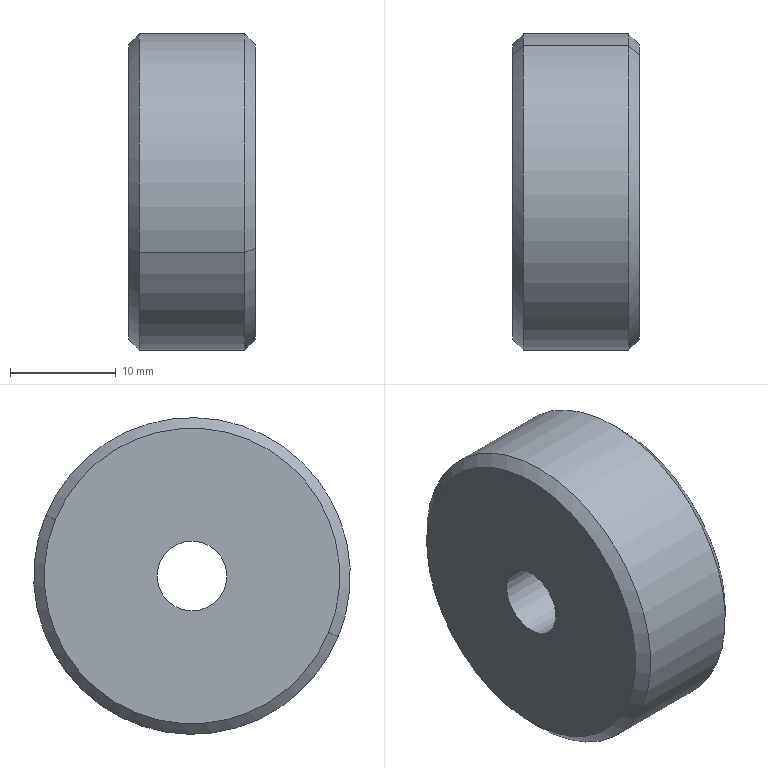Component | SolidWorks | JJDJR-3060-E-005-1 | 1 solid | 13 faces | box 12 x 30 x 30 mm | volume 7427 mm3 | cylinder 6 | cone 4 | plane 3 | commonest cylinder face diameters 12 x2 6.6 x2 30 x2 | material Tungsten Alloy
build123d program:
from build123d import *

# Parameters (mm, degrees)
SKETCH1_W                                           = 12
SKETCH1_H                                           = 15
CHAMFER1_SIZE                                       = 1
CYLINDRICAL_COUNTERSUNK_HOLE_FOR_M6_HEX_D           = 6.6
CYLINDRICAL_COUNTERSUNK_HOLE_FOR_M6_HEX_CBORE_D     = 12
CYLINDRICAL_COUNTERSUNK_HOLE_FOR_M6_HEX_CBORE_DEPTH = 7


with BuildPart() as part:
    # Sketch1 → Revolve1 (revolve)
    with BuildSketch(Plane.XY, mode=Mode.PRIVATE) as revolve1_sk:
        with Locations((6, 7.5)):
            Rectangle(SKETCH1_W, SKETCH1_H)
    revolve(revolve1_sk.sketch.rotate(Axis((-79.76, 0, 0), (1, 0, 0)), 90), axis=Axis((-79.76, 0, 0), (1, 0, 0)))

    # Chamfer1
    chamfer1_edges = [part.edges().sort_by_distance(p)[0] for p in [
        (0, 0, -15),
        (12, 0, -15),
    ]]
    chamfer(chamfer1_edges, length=CHAMFER1_SIZE)

    # Cylindrical Countersunk Hole for M6 Hex (through all)
    with Locations(Plane.ZY):
        with Locations((0, 0)):
            CounterBoreHole(CYLINDRICAL_COUNTERSUNK_HOLE_FOR_M6_HEX_D / 2, CYLINDRICAL_COUNTERSUNK_HOLE_FOR_M6_HEX_CBORE_D / 2, CYLINDRICAL_COUNTERSUNK_HOLE_FOR_M6_HEX_CBORE_DEPTH)


solid = part.part

# Placed as in the assembly
solid = solid.moved(Location((113.41, -29.263, -16.52), (-180, 0, 180)))
STEP:
#1=COLOUR_RGB('',0.7922,0.8196,0.9333);
#2=FILL_AREA_STYLE_COLOUR('',#1);
#3=FILL_AREA_STYLE('',(#2));
#4=SURFACE_STYLE_FILL_AREA(#3);
#5=SURFACE_SIDE_STYLE('',(#4));
#6=SURFACE_STYLE_USAGE(.BOTH.,#5);
#7=PRESENTATION_STYLE_ASSIGNMENT((#6));
#8=CARTESIAN_POINT('',(4.189,-1.37,-0.7406));
#9=VERTEX_POINT('',#8);
#10=CARTESIAN_POINT('',(4.189,-0.9338,-0.5602));
#11=VERTEX_POINT('',#10);
#12=CARTESIAN_POINT('',(4.189,-1.152,-0.6504));
#13=DIRECTION('',(1.,0.,0.));
#14=DIRECTION('',(0.,0.9242,0.3818));
#15=AXIS2_PLACEMENT_3D('',#12,#13,#14);
#16=CIRCLE('',#15,0.2362);
#17=EDGE_CURVE('',#9,#11,#16,.T.);
#18=ORIENTED_EDGE('',*,*,#17,.F.);
#19=CARTESIAN_POINT('',(4.465,-1.37,-0.7406));
#20=VERTEX_POINT('',#19);
#21=CARTESIAN_POINT('',(4.465,-1.37,-0.7406));
#22=DIRECTION('',(1.,0.,0.));
#23=VECTOR('',#22,39.37);
#24=LINE('',#21,#23);
#25=EDGE_CURVE('',#9,#20,#24,.T.);
#26=ORIENTED_EDGE('',*,*,#25,.T.);
#27=CARTESIAN_POINT('',(4.465,-0.9338,-0.5602));
#28=VERTEX_POINT('',#27);
#29=CARTESIAN_POINT('',(4.465,-1.152,-0.6504));
#30=DIRECTION('',(1.,0.,0.));
#31=DIRECTION('',(0.,0.9242,0.3818));
#32=AXIS2_PLACEMENT_3D('',#29,#30,#31);
#33=CIRCLE('',#32,0.2362);
#34=EDGE_CURVE('',#20,#28,#33,.T.);
#35=ORIENTED_EDGE('',*,*,#34,.T.);
#36=CARTESIAN_POINT('',(4.465,-0.9338,-0.5602));
#37=DIRECTION('',(1.,0.,0.));
#38=VECTOR('',#37,39.37);
#39=LINE('',#36,#38);
#40=EDGE_CURVE('',#11,#28,#39,.T.);
#41=ORIENTED_EDGE('',*,*,#40,.F.);
#42=EDGE_LOOP('',(#18,#26,#35,#41));
#43=FACE_OUTER_BOUND('',#42,.T.);
#44=CARTESIAN_POINT('',(4.465,-1.152,-0.6504));
#45=DIRECTION('',(1.,0.,0.));
#46=DIRECTION('',(0.,0.9242,0.3818));
#47=AXIS2_PLACEMENT_3D('',#44,#45,#46);
#48=CYLINDRICAL_SURFACE('',#47,0.2362);
#49=ADVANCED_FACE('',(#43),#48,.F.);
#50=CARTESIAN_POINT('',(3.993,-1.272,-0.7));
#51=VERTEX_POINT('',#50);
#52=CARTESIAN_POINT('',(3.993,-1.032,-0.6008));
#53=VERTEX_POINT('',#52);
#54=CARTESIAN_POINT('',(3.993,-1.152,-0.6504));
#55=DIRECTION('',(1.,0.,0.));
#56=DIRECTION('',(0.,0.9242,0.3818));
#57=AXIS2_PLACEMENT_3D('',#54,#55,#56);
#58=CIRCLE('',#57,0.1299);
#59=EDGE_CURVE('',#51,#53,#58,.T.);
#60=ORIENTED_EDGE('',*,*,#59,.F.);
#61=CARTESIAN_POINT('',(4.189,-1.272,-0.7));
#62=VERTEX_POINT('',#61);
#63=CARTESIAN_POINT('',(4.465,-1.272,-0.7));
#64=DIRECTION('',(1.,0.,0.));
#65=VECTOR('',#64,39.37);
#66=LINE('',#63,#65);
#67=EDGE_CURVE('',#51,#62,#66,.T.);
#68=ORIENTED_EDGE('',*,*,#67,.T.);
#69=CARTESIAN_POINT('',(4.189,-1.032,-0.6008));
#70=VERTEX_POINT('',#69);
#71=CARTESIAN_POINT('',(4.189,-1.152,-0.6504));
#72=DIRECTION('',(1.,0.,0.));
#73=DIRECTION('',(0.,0.9242,0.3818));
#74=AXIS2_PLACEMENT_3D('',#71,#72,#73);
#75=CIRCLE('',#74,0.1299);
#76=EDGE_CURVE('',#62,#70,#75,.T.);
#77=ORIENTED_EDGE('',*,*,#76,.T.);
#78=CARTESIAN_POINT('',(4.465,-1.032,-0.6008));
#79=DIRECTION('',(1.,0.,0.));
#80=VECTOR('',#79,39.37);
#81=LINE('',#78,#80);
#82=EDGE_CURVE('',#53,#70,#81,.T.);
#83=ORIENTED_EDGE('',*,*,#82,.F.);
#84=EDGE_LOOP('',(#60,#68,#77,#83));
#85=FACE_OUTER_BOUND('',#84,.T.);
#86=CARTESIAN_POINT('',(4.465,-1.152,-0.6504));
#87=DIRECTION('',(1.,0.,0.));
#88=DIRECTION('',(0.,0.9242,0.3818));
#89=AXIS2_PLACEMENT_3D('',#86,#87,#88);
#90=CYLINDRICAL_SURFACE('',#89,0.1299);
#91=ADVANCED_FACE('',(#85),#90,.F.);
#92=CARTESIAN_POINT('',(4.465,-0.6427,-0.4399));
#93=VERTEX_POINT('',#92);
#94=CARTESIAN_POINT('',(4.465,-1.661,-0.8609));
#95=VERTEX_POINT('',#94);
#96=CARTESIAN_POINT('',(4.465,-1.152,-0.6504));
#97=DIRECTION('',(1.,0.,0.));
#98=DIRECTION('',(0.,-0.9242,-0.3818));
#99=AXIS2_PLACEMENT_3D('',#96,#97,#98);
#100=CIRCLE('',#99,0.5512);
#101=EDGE_CURVE('',#93,#95,#100,.T.);
#102=ORIENTED_EDGE('',*,*,#101,.F.);
#103=CARTESIAN_POINT('',(4.426,-0.6063,-0.4249));
#104=VERTEX_POINT('',#103);
#105=CARTESIAN_POINT('',(4.465,-0.6427,-0.4399));
#106=DIRECTION('',(-0.7071,0.6535,0.27));
#107=VECTOR('',#106,39.37);
#108=LINE('',#105,#107);
#109=EDGE_CURVE('',#93,#104,#108,.T.);
#110=ORIENTED_EDGE('',*,*,#109,.T.);
#111=CARTESIAN_POINT('',(4.426,-1.698,-0.8759));
#112=VERTEX_POINT('',#111);
#113=CARTESIAN_POINT('',(4.426,-1.152,-0.6504));
#114=DIRECTION('',(-1.,0.,0.));
#115=DIRECTION('',(0.,-0.9242,-0.3818));
#116=AXIS2_PLACEMENT_3D('',#113,#114,#115);
#117=CIRCLE('',#116,0.5906);
#118=EDGE_CURVE('',#112,#104,#117,.T.);
#119=ORIENTED_EDGE('',*,*,#118,.F.);
#120=CARTESIAN_POINT('',(4.465,-1.661,-0.8609));
#121=DIRECTION('',(-0.7071,-0.6535,-0.27));
#122=VECTOR('',#121,39.37);
#123=LINE('',#120,#122);
#124=EDGE_CURVE('',#95,#112,#123,.T.);
#125=ORIENTED_EDGE('',*,*,#124,.F.);
#126=EDGE_LOOP('',(#102,#110,#119,#125));
#127=FACE_OUTER_BOUND('',#126,.T.);
#128=CARTESIAN_POINT('',(4.465,-1.152,-0.6504));
#129=DIRECTION('',(-1.,0.,0.));
#130=DIRECTION('',(0.,-0.9242,-0.3818));
#131=AXIS2_PLACEMENT_3D('',#128,#129,#130);
#132=CONICAL_SURFACE('',#131,0.5512,0.7854);
#133=ADVANCED_FACE('',(#127),#132,.T.);
#134=CARTESIAN_POINT('',(3.993,-1.661,-0.8609));
#135=VERTEX_POINT('',#134);
#136=CARTESIAN_POINT('',(3.993,-0.6427,-0.4399));
#137=VERTEX_POINT('',#136);
#138=CARTESIAN_POINT('',(3.993,-1.152,-0.6504));
#139=DIRECTION('',(-1.,0.,0.));
#140=DIRECTION('',(0.,0.9242,0.3818));
#141=AXIS2_PLACEMENT_3D('',#138,#139,#140);
#142=CIRCLE('',#141,0.5512);
#143=EDGE_CURVE('',#135,#137,#142,.T.);
#144=ORIENTED_EDGE('',*,*,#143,.F.);
#145=CARTESIAN_POINT('',(4.032,-1.698,-0.8759));
#146=VERTEX_POINT('',#145);
#147=CARTESIAN_POINT('',(4.032,-1.698,-0.8759));
#148=DIRECTION('',(0.7071,-0.6535,-0.27));
#149=VECTOR('',#148,39.37);
#150=LINE('',#147,#149);
#151=EDGE_CURVE('',#135,#146,#150,.T.);
#152=ORIENTED_EDGE('',*,*,#151,.T.);
#153=CARTESIAN_POINT('',(4.032,-0.6063,-0.4249));
#154=VERTEX_POINT('',#153);
#155=CARTESIAN_POINT('',(4.032,-1.152,-0.6504));
#156=DIRECTION('',(1.,0.,0.));
#157=DIRECTION('',(0.,0.9242,0.3818));
#158=AXIS2_PLACEMENT_3D('',#155,#156,#157);
#159=CIRCLE('',#158,0.5906);
#160=EDGE_CURVE('',#154,#146,#159,.T.);
#161=ORIENTED_EDGE('',*,*,#160,.F.);
#162=CARTESIAN_POINT('',(4.032,-0.6063,-0.4249));
#163=DIRECTION('',(0.7071,0.6535,0.27));
#164=VECTOR('',#163,39.37);
#165=LINE('',#162,#164);
#166=EDGE_CURVE('',#137,#154,#165,.T.);
#167=ORIENTED_EDGE('',*,*,#166,.F.);
#168=EDGE_LOOP('',(#144,#152,#161,#167));
#169=FACE_OUTER_BOUND('',#168,.T.);
#170=CARTESIAN_POINT('',(4.032,-1.152,-0.6504));
#171=DIRECTION('',(1.,0.,0.));
#172=DIRECTION('',(0.,0.9242,0.3818));
#173=AXIS2_PLACEMENT_3D('',#170,#171,#172);
#174=CONICAL_SURFACE('',#173,0.5906,0.7854);
#175=ADVANCED_FACE('',(#169),#174,.T.);
#176=ORIENTED_EDGE('',*,*,#160,.T.);
#177=CARTESIAN_POINT('',(7.605,-1.698,-0.8759));
#178=DIRECTION('',(1.,0.,0.));
#179=VECTOR('',#178,39.37);
#180=LINE('',#177,#179);
#181=EDGE_CURVE('',#146,#112,#180,.T.);
#182=ORIENTED_EDGE('',*,*,#181,.T.);
#183=ORIENTED_EDGE('',*,*,#118,.T.);
#184=CARTESIAN_POINT('',(7.605,-0.6063,-0.4249));
#185=DIRECTION('',(1.,0.,0.));
#186=VECTOR('',#185,39.37);
#187=LINE('',#184,#186);
#188=EDGE_CURVE('',#154,#104,#187,.T.);
#189=ORIENTED_EDGE('',*,*,#188,.F.);
#190=EDGE_LOOP('',(#176,#182,#183,#189));
#191=FACE_OUTER_BOUND('',#190,.T.);
#192=CARTESIAN_POINT('',(7.605,-1.152,-0.6504));
#193=DIRECTION('',(1.,0.,0.));
#194=DIRECTION('',(0.,0.9242,0.3818));
#195=AXIS2_PLACEMENT_3D('',#192,#193,#194);
#196=CYLINDRICAL_SURFACE('',#195,0.5906);
#197=ADVANCED_FACE('',(#191),#196,.T.);
#198=CARTESIAN_POINT('',(4.465,-1.152,-0.6504));
#199=DIRECTION('',(1.,0.,0.));
#200=DIRECTION('',(0.,0.9242,0.3818));
#201=AXIS2_PLACEMENT_3D('',#198,#199,#200);
#202=CIRCLE('',#201,0.2362);
#203=EDGE_CURVE('',#28,#20,#202,.T.);
#204=ORIENTED_EDGE('',*,*,#203,.F.);
#205=ORIENTED_EDGE('',*,*,#34,.F.);
#206=EDGE_LOOP('',(#204,#205));
#207=FACE_BOUND('',#206,.T.);
#208=CARTESIAN_POINT('',(4.465,-1.152,-0.6504));
#209=DIRECTION('',(1.,0.,0.));
#210=DIRECTION('',(0.,-0.9242,-0.3818));
#211=AXIS2_PLACEMENT_3D('',#208,#209,#210);
#212=CIRCLE('',#211,0.5512);
#213=EDGE_CURVE('',#95,#93,#212,.T.);
#214=ORIENTED_EDGE('',*,*,#213,.T.);
#215=ORIENTED_EDGE('',*,*,#101,.T.);
#216=EDGE_LOOP('',(#214,#215));
#217=FACE_OUTER_BOUND('',#216,.T.);
#218=CARTESIAN_POINT('',(4.465,-1.378,-0.1046));
#219=DIRECTION('',(-1.,0.,0.));
#220=DIRECTION('',(0.,-0.9242,-0.3818));
#221=AXIS2_PLACEMENT_3D('',#218,#219,#220);
#222=PLANE('',#221);
#223=ADVANCED_FACE('',(#207,#217),#222,.F.);
#224=CARTESIAN_POINT('',(3.993,-1.152,-0.6504));
#225=DIRECTION('',(1.,0.,0.));
#226=DIRECTION('',(0.,0.9242,0.3818));
#227=AXIS2_PLACEMENT_3D('',#224,#225,#226);
#228=CIRCLE('',#227,0.1299);
#229=EDGE_CURVE('',#53,#51,#228,.T.);
#230=ORIENTED_EDGE('',*,*,#229,.T.);
#231=ORIENTED_EDGE('',*,*,#59,.T.);
#232=EDGE_LOOP('',(#230,#231));
#233=FACE_BOUND('',#232,.T.);
#234=CARTESIAN_POINT('',(3.993,-1.152,-0.6504));
#235=DIRECTION('',(-1.,0.,0.));
#236=DIRECTION('',(0.,0.9242,0.3818));
#237=AXIS2_PLACEMENT_3D('',#234,#235,#236);
#238=CIRCLE('',#237,0.5512);
#239=EDGE_CURVE('',#137,#135,#238,.T.);
#240=ORIENTED_EDGE('',*,*,#239,.T.);
#241=ORIENTED_EDGE('',*,*,#143,.T.);
#242=EDGE_LOOP('',(#240,#241));
#243=FACE_OUTER_BOUND('',#242,.T.);
#244=CARTESIAN_POINT('',(3.993,-1.152,-0.6504));
#245=DIRECTION('',(1.,0.,0.));
#246=DIRECTION('',(0.,0.9242,0.3818));
#247=AXIS2_PLACEMENT_3D('',#244,#245,#246);
#248=PLANE('',#247);
#249=ADVANCED_FACE('',(#233,#243),#248,.F.);
#250=ORIENTED_EDGE('',*,*,#181,.F.);
#251=CARTESIAN_POINT('',(4.032,-1.152,-0.6504));
#252=DIRECTION('',(1.,0.,0.));
#253=DIRECTION('',(0.,0.9242,0.3818));
#254=AXIS2_PLACEMENT_3D('',#251,#252,#253);
#255=CIRCLE('',#254,0.5906);
#256=EDGE_CURVE('',#146,#154,#255,.T.);
#257=ORIENTED_EDGE('',*,*,#256,.T.);
#258=ORIENTED_EDGE('',*,*,#188,.T.);
#259=CARTESIAN_POINT('',(4.426,-1.152,-0.6504));
#260=DIRECTION('',(-1.,0.,0.));
#261=DIRECTION('',(0.,-0.9242,-0.3818));
#262=AXIS2_PLACEMENT_3D('',#259,#260,#261);
#263=CIRCLE('',#262,0.5906);
#264=EDGE_CURVE('',#104,#112,#263,.T.);
#265=ORIENTED_EDGE('',*,*,#264,.T.);
#266=EDGE_LOOP('',(#250,#257,#258,#265));
#267=FACE_OUTER_BOUND('',#266,.T.);
#268=CARTESIAN_POINT('',(7.605,-1.152,-0.6504));
#269=DIRECTION('',(1.,0.,0.));
#270=DIRECTION('',(0.,0.9242,0.3818));
#271=AXIS2_PLACEMENT_3D('',#268,#269,#270);
#272=CYLINDRICAL_SURFACE('',#271,0.5906);
#273=ADVANCED_FACE('',(#267),#272,.T.);
#274=ORIENTED_EDGE('',*,*,#151,.F.);
#275=ORIENTED_EDGE('',*,*,#239,.F.);
#276=ORIENTED_EDGE('',*,*,#166,.T.);
#277=ORIENTED_EDGE('',*,*,#256,.F.);
#278=EDGE_LOOP('',(#274,#275,#276,#277));
#279=FACE_OUTER_BOUND('',#278,.T.);
#280=CARTESIAN_POINT('',(4.032,-1.152,-0.6504));
#281=DIRECTION('',(1.,0.,0.));
#282=DIRECTION('',(0.,0.9242,0.3818));
#283=AXIS2_PLACEMENT_3D('',#280,#281,#282);
#284=CONICAL_SURFACE('',#283,0.5906,0.7854);
#285=ADVANCED_FACE('',(#279),#284,.T.);
#286=ORIENTED_EDGE('',*,*,#109,.F.);
#287=ORIENTED_EDGE('',*,*,#213,.F.);
#288=ORIENTED_EDGE('',*,*,#124,.T.);
#289=ORIENTED_EDGE('',*,*,#264,.F.);
#290=EDGE_LOOP('',(#286,#287,#288,#289));
#291=FACE_OUTER_BOUND('',#290,.T.);
#292=CARTESIAN_POINT('',(4.465,-1.152,-0.6504));
#293=DIRECTION('',(-1.,0.,0.));
#294=DIRECTION('',(0.,-0.9242,-0.3818));
#295=AXIS2_PLACEMENT_3D('',#292,#293,#294);
#296=CONICAL_SURFACE('',#295,0.5512,0.7854);
#297=ADVANCED_FACE('',(#291),#296,.T.);
#298=ORIENTED_EDGE('',*,*,#67,.F.);
#299=ORIENTED_EDGE('',*,*,#229,.F.);
#300=ORIENTED_EDGE('',*,*,#82,.T.);
#301=CARTESIAN_POINT('',(4.189,-1.152,-0.6504));
#302=DIRECTION('',(1.,0.,0.));
#303=DIRECTION('',(0.,0.9242,0.3818));
#304=AXIS2_PLACEMENT_3D('',#301,#302,#303);
#305=CIRCLE('',#304,0.1299);
#306=EDGE_CURVE('',#70,#62,#305,.T.);
#307=ORIENTED_EDGE('',*,*,#306,.T.);
#308=EDGE_LOOP('',(#298,#299,#300,#307));
#309=FACE_OUTER_BOUND('',#308,.T.);
#310=CARTESIAN_POINT('',(4.465,-1.152,-0.6504));
#311=DIRECTION('',(1.,0.,0.));
#312=DIRECTION('',(0.,0.9242,0.3818));
#313=AXIS2_PLACEMENT_3D('',#310,#311,#312);
#314=CYLINDRICAL_SURFACE('',#313,0.1299);
#315=ADVANCED_FACE('',(#309),#314,.F.);
#316=ORIENTED_EDGE('',*,*,#306,.F.);
#317=ORIENTED_EDGE('',*,*,#76,.F.);
#318=EDGE_LOOP('',(#316,#317));
#319=FACE_BOUND('',#318,.T.);
#320=CARTESIAN_POINT('',(4.189,-1.152,-0.6504));
#321=DIRECTION('',(1.,0.,0.));
#322=DIRECTION('',(0.,0.9242,0.3818));
#323=AXIS2_PLACEMENT_3D('',#320,#321,#322);
#324=CIRCLE('',#323,0.2362);
#325=EDGE_CURVE('',#11,#9,#324,.T.);
#326=ORIENTED_EDGE('',*,*,#325,.T.);
#327=ORIENTED_EDGE('',*,*,#17,.T.);
#328=EDGE_LOOP('',(#326,#327));
#329=FACE_OUTER_BOUND('',#328,.T.);
#330=CARTESIAN_POINT('',(4.189,-1.202,-0.5303));
#331=DIRECTION('',(-1.,0.,0.));
#332=DIRECTION('',(0.,-0.9242,-0.3818));
#333=AXIS2_PLACEMENT_3D('',#330,#331,#332);
#334=PLANE('',#333);
#335=ADVANCED_FACE('',(#319,#329),#334,.F.);
#336=ORIENTED_EDGE('',*,*,#25,.F.);
#337=ORIENTED_EDGE('',*,*,#325,.F.);
#338=ORIENTED_EDGE('',*,*,#40,.T.);
#339=ORIENTED_EDGE('',*,*,#203,.T.);
#340=EDGE_LOOP('',(#336,#337,#338,#339));
#341=FACE_OUTER_BOUND('',#340,.T.);
#342=CARTESIAN_POINT('',(4.465,-1.152,-0.6504));
#343=DIRECTION('',(1.,0.,0.));
#344=DIRECTION('',(0.,0.9242,0.3818));
#345=AXIS2_PLACEMENT_3D('',#342,#343,#344);
#346=CYLINDRICAL_SURFACE('',#345,0.2362);
#347=ADVANCED_FACE('',(#341),#346,.F.);
#348=CLOSED_SHELL('',(#49,#91,#133,#175,#197,#223,#249,#273,#285,#297,#315,#335,#347));
#349=MANIFOLD_SOLID_BREP('',#348);
#350=STYLED_ITEM('',(#7),#349);
#351=(LENGTH_UNIT()NAMED_UNIT(*)SI_UNIT($,.METRE.));
#352=LENGTH_MEASURE_WITH_UNIT(LENGTH_MEASURE(0.0254),#351);
#353=DIMENSIONAL_EXPONENTS(1.,0.,0.,0.,0.,0.,0.);
#354=(CONVERSION_BASED_UNIT('',#352)LENGTH_UNIT()NAMED_UNIT(#353));
#355=UNCERTAINTY_MEASURE_WITH_UNIT(LENGTH_MEASURE(0.00001),#354,'','');
#356=(NAMED_UNIT(*)PLANE_ANGLE_UNIT()SI_UNIT($,.RADIAN.));
#357=(NAMED_UNIT(*)SI_UNIT($,.STERADIAN.)SOLID_ANGLE_UNIT());
#358=(GEOMETRIC_REPRESENTATION_CONTEXT(3)GLOBAL_UNCERTAINTY_ASSIGNED_CONTEXT((#355))GLOBAL_UNIT_ASSIGNED_CONTEXT((#354,#356,#357))REPRESENTATION_CONTEXT('',''));
#359=MECHANICAL_DESIGN_GEOMETRIC_PRESENTATION_REPRESENTATION('',(#350),#358);
#360=PRESENTATION_LAYER_ASSIGNMENT('','',(#350));
#361=CARTESIAN_POINT('',(0.,0.,0.));
#362=DIRECTION('',(0.,0.,1.));
#363=DIRECTION('',(1.,0.,0.));
#364=AXIS2_PLACEMENT_3D('',#361,#362,#363);
#365=(LENGTH_UNIT()NAMED_UNIT(*)SI_UNIT($,.METRE.));
#366=LENGTH_MEASURE_WITH_UNIT(LENGTH_MEASURE(0.0254),#365);
#367=DIMENSIONAL_EXPONENTS(1.,0.,0.,0.,0.,0.,0.);
#368=(CONVERSION_BASED_UNIT('',#366)LENGTH_UNIT()NAMED_UNIT(#367));
#369=UNCERTAINTY_MEASURE_WITH_UNIT(LENGTH_MEASURE(0.00001),#368,'','');
#370=(NAMED_UNIT(*)PLANE_ANGLE_UNIT()SI_UNIT($,.RADIAN.));
#371=(NAMED_UNIT(*)SI_UNIT($,.STERADIAN.)SOLID_ANGLE_UNIT());
#372=(GEOMETRIC_REPRESENTATION_CONTEXT(3)GLOBAL_UNCERTAINTY_ASSIGNED_CONTEXT((#369))GLOBAL_UNIT_ASSIGNED_CONTEXT((#368,#370,#371))REPRESENTATION_CONTEXT('',''));
#373=ADVANCED_BREP_SHAPE_REPRESENTATION('',(#349,#364),#372);